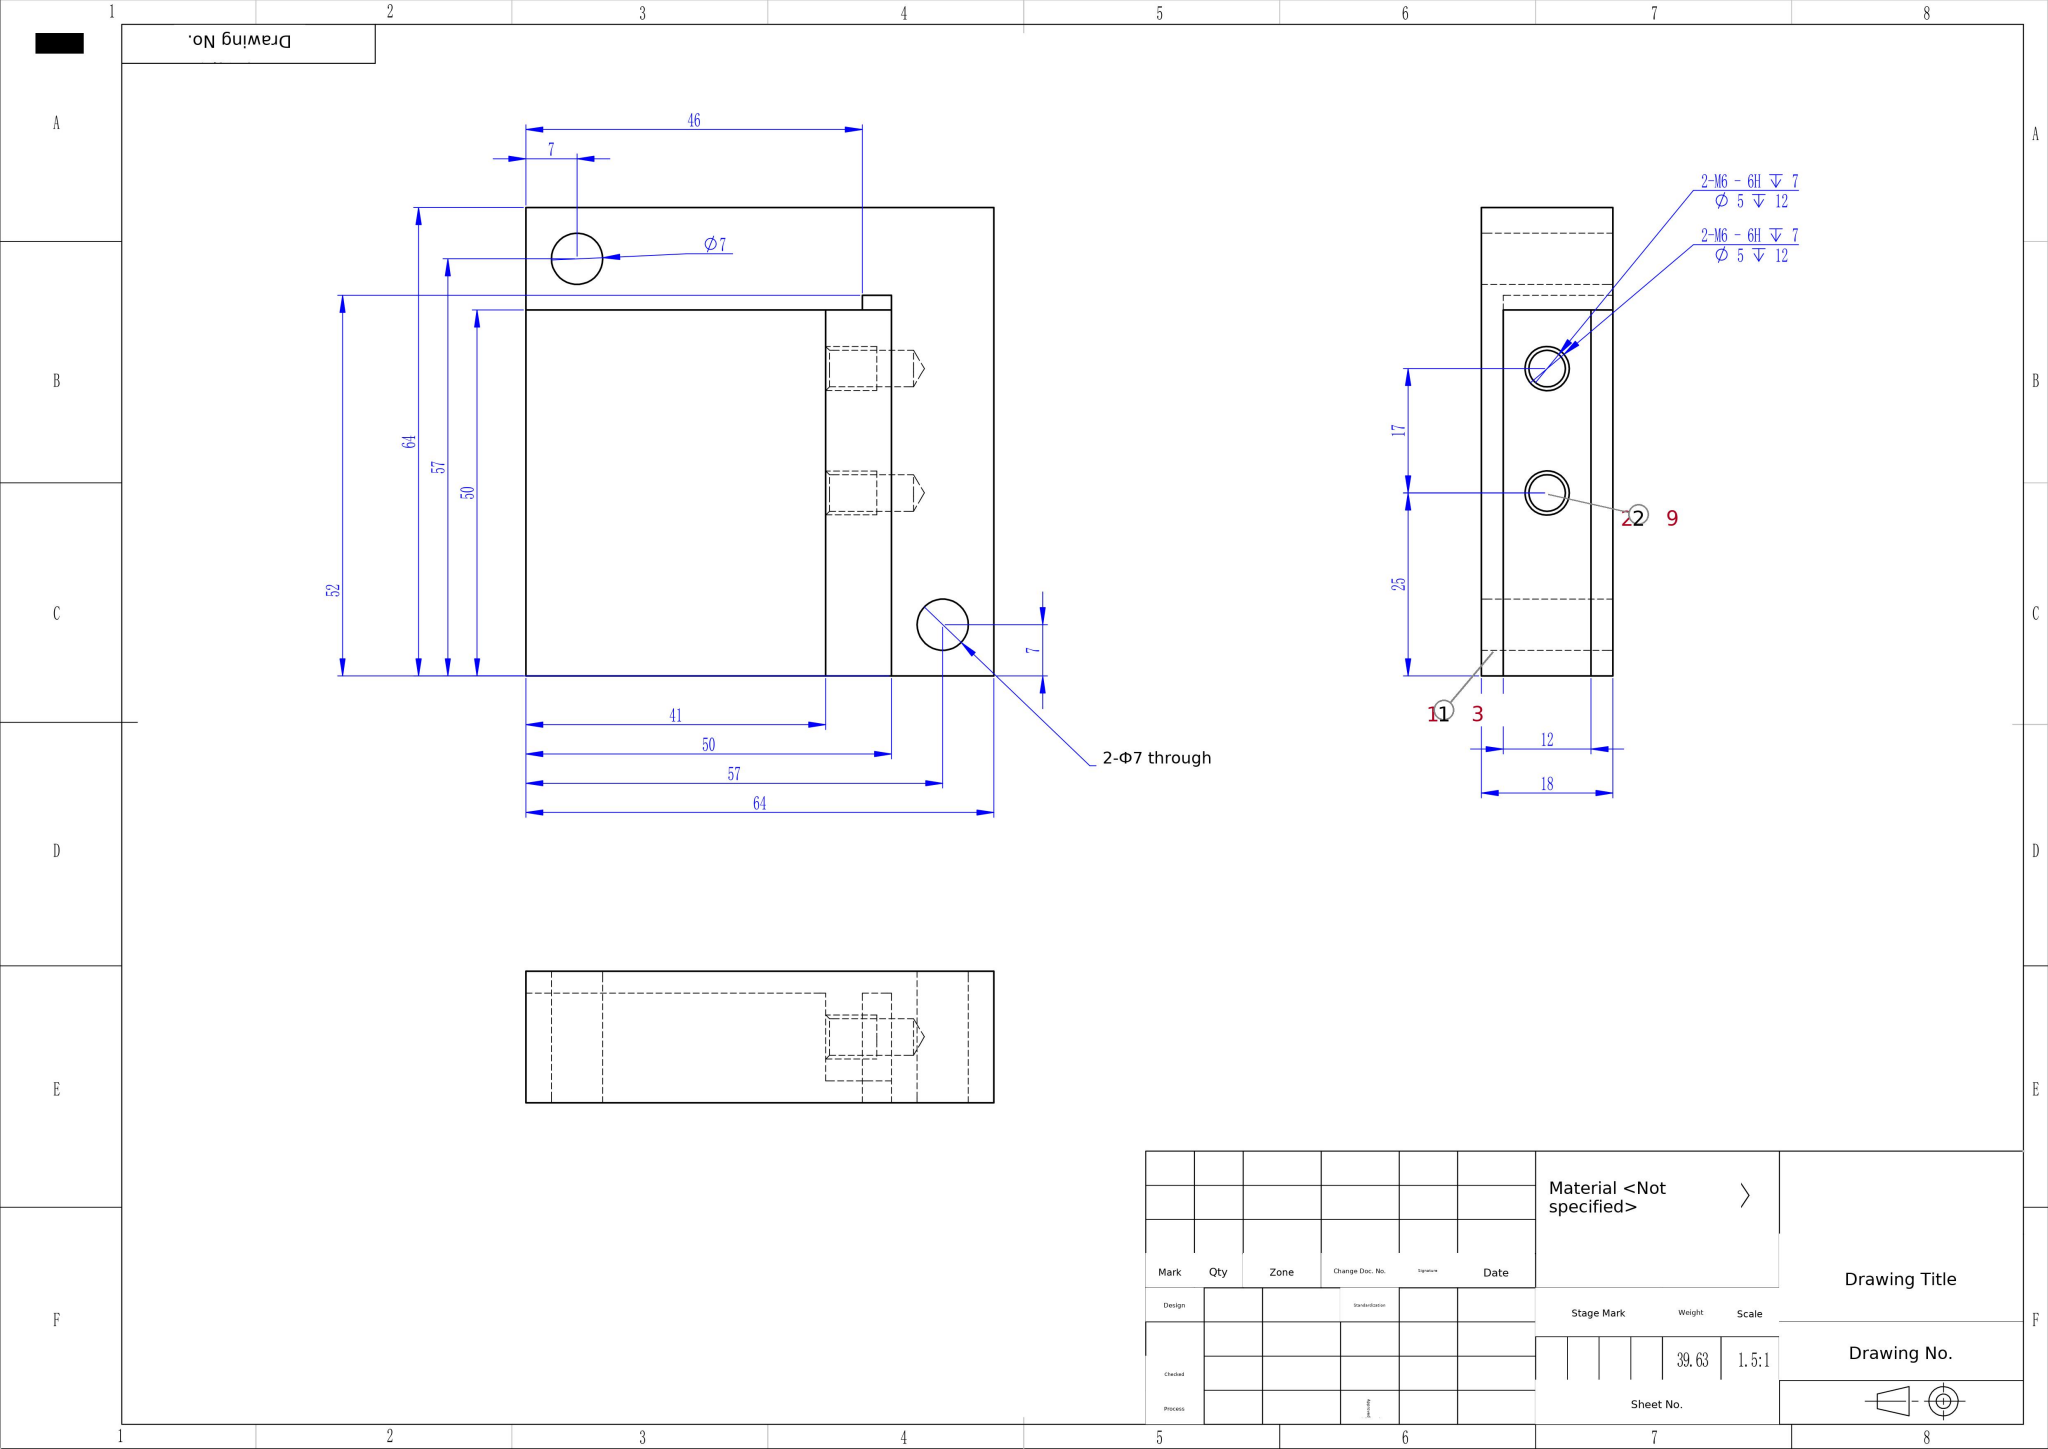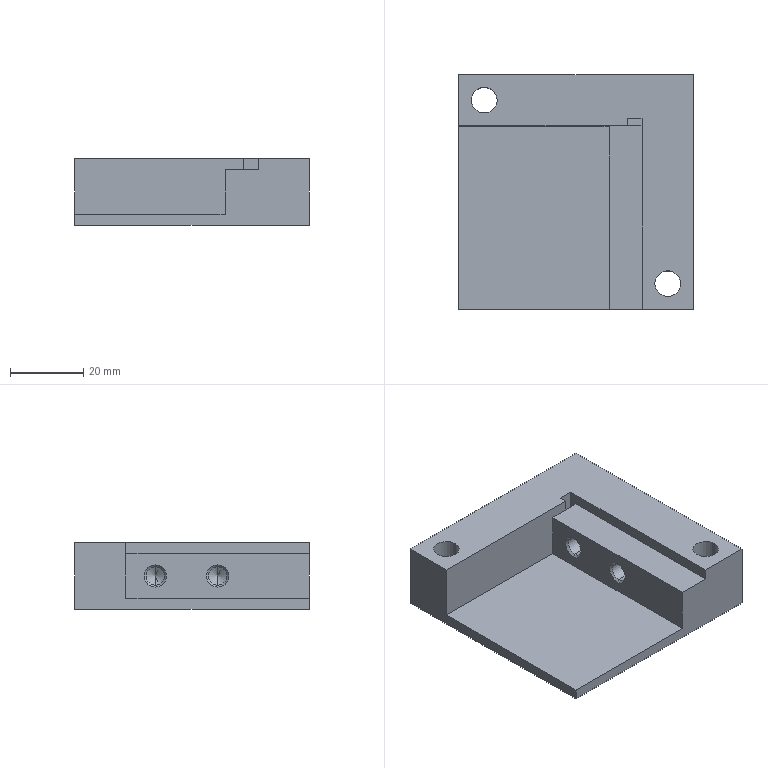Part | SolidWorks | mm | 1 solid | 31 faces | box 64 x 64 x 18 mm | volume 39627 mm3 | plane 15 | cone 8 | cylinder 8 | commonest cylinder face diameters 5 x4 7 x4
build123d program:
from build123d import *

# Parameters (mm, degrees)
SKETCH1_W                   = 64
SKETCH1_H                   = 64
BOSS_EXTRUDE1_DEPTH         = 3
BOSS_EXTRUDE2_DEPTH         = 15
CUT_EXTRUDE1_REACH          = 50.703
SKETCH4_R                   = 3.5
SKETCH6_W                   = 9
SKETCH6_H                   = 12
BOSS_EXTRUDE3_DEPTH         = 50
M6_TAPPED_HOLE1_D           = 5
M6_TAPPED_HOLE1_DEPTH       = 12
M6_TAPPED_HOLE1_CSINK_D     = 6.05
M6_TAPPED_HOLE1_CSINK_ANGLE = 90
M6_TAPPED_HOLE1_TIP         = 1.502


with BuildPart() as part:
    # Sketch1 → Boss-Extrude1 (new body)
    with BuildSketch(Plane.XY):
        Rectangle(SKETCH1_W, SKETCH1_H)
    extrude(amount=BOSS_EXTRUDE1_DEPTH)

    # Sketch3 → Boss-Extrude2 (add)
    with BuildSketch(Plane.XY.offset(3)):
        Polygon((-32, 32), (32, 32), (32, -32), (18, -32), (18, 20), (14, 20), (14, 18), (-32, 18), align=None)
    extrude(amount=BOSS_EXTRUDE2_DEPTH)

    # Sketch4 → Cut-Extrude1 (cut, up to next)
    with BuildSketch(Plane.XY.offset(18), mode=Mode.PRIVATE) as cut_extrude1_sk1:
        with Locations((-25, 25)):
            Circle(SKETCH4_R)
    cut_extrude1_tool1 = extrude(cut_extrude1_sk1.sketch, amount=-CUT_EXTRUDE1_REACH, mode=Mode.PRIVATE) & part.part
    # Sketch4 → Cut-Extrude1 (cut, up to next)
    with BuildSketch(Plane.XY.offset(18), mode=Mode.PRIVATE) as cut_extrude1_sk2:
        with Locations((25, -25)):
            Circle(SKETCH4_R)
    cut_extrude1_tool2 = extrude(cut_extrude1_sk2.sketch, amount=-CUT_EXTRUDE1_REACH, mode=Mode.PRIVATE) & part.part
    add(cut_extrude1_tool1.solids().sort_by_distance((-25, 25, 18))[0], mode=Mode.SUBTRACT)
    add(cut_extrude1_tool2.solids().sort_by_distance((25, -25, 18))[0], mode=Mode.SUBTRACT)

    # Sketch6 → Boss-Extrude3 (add)
    with BuildSketch(Plane.XZ.offset(32)):
        with Locations((13.5, 9)):
            Rectangle(SKETCH6_W, SKETCH6_H)
    extrude(amount=-BOSS_EXTRUDE3_DEPTH)

    # M6 Tapped Hole1
    with Locations(Plane.ZY.offset(-9)):
        with Locations((9, 10), (9, -7)):
            CounterSinkHole(M6_TAPPED_HOLE1_D / 2, M6_TAPPED_HOLE1_CSINK_D / 2, depth=M6_TAPPED_HOLE1_DEPTH, counter_sink_angle=M6_TAPPED_HOLE1_CSINK_ANGLE)
            with Locations((0, 0, -(M6_TAPPED_HOLE1_DEPTH + M6_TAPPED_HOLE1_TIP / 2))):  # 118° drill point
                Cone(0, M6_TAPPED_HOLE1_D / 2, M6_TAPPED_HOLE1_TIP, mode=Mode.SUBTRACT)


solid = part.part
STEP:
#1=CARTESIAN_POINT('',(9.525,10.,6.5));
#2=VERTEX_POINT('',#1);
#3=CARTESIAN_POINT('',(9.525,10.,11.5));
#4=VERTEX_POINT('',#3);
#5=CARTESIAN_POINT('',(9.525,10.,9.));
#6=DIRECTION('',(-1.,0.,-0.));
#7=DIRECTION('',(0.,0.,1.));
#8=AXIS2_PLACEMENT_3D('',#5,#6,#7);
#9=CIRCLE('',#8,2.5);
#10=EDGE_CURVE('',#2,#4,#9,.T.);
#11=ORIENTED_EDGE('',*,*,#10,.F.);
#12=CARTESIAN_POINT('',(9.,10.,5.975));
#13=VERTEX_POINT('',#12);
#14=CARTESIAN_POINT('',(9.,10.,5.975));
#15=DIRECTION('',(-0.7071,0.,-0.7071));
#16=VECTOR('',#15,1000.);
#17=LINE('',#14,#16);
#18=EDGE_CURVE('',#2,#13,#17,.T.);
#19=ORIENTED_EDGE('',*,*,#18,.T.);
#20=CARTESIAN_POINT('',(9.,10.,12.025));
#21=VERTEX_POINT('',#20);
#22=CARTESIAN_POINT('',(9.,10.,9.));
#23=DIRECTION('',(-1.,0.,-0.));
#24=DIRECTION('',(0.,0.,1.));
#25=AXIS2_PLACEMENT_3D('',#22,#23,#24);
#26=CIRCLE('',#25,3.025);
#27=EDGE_CURVE('',#13,#21,#26,.T.);
#28=ORIENTED_EDGE('',*,*,#27,.T.);
#29=CARTESIAN_POINT('',(9.,10.,12.025));
#30=DIRECTION('',(-0.7071,0.,0.7071));
#31=VECTOR('',#30,1000.);
#32=LINE('',#29,#31);
#33=EDGE_CURVE('',#4,#21,#32,.T.);
#34=ORIENTED_EDGE('',*,*,#33,.F.);
#35=EDGE_LOOP('',(#11,#19,#28,#34));
#36=FACE_OUTER_BOUND('',#35,.T.);
#37=CARTESIAN_POINT('',(9.,10.,9.));
#38=DIRECTION('',(-1.,0.,-0.));
#39=DIRECTION('',(0.,0.,1.));
#40=AXIS2_PLACEMENT_3D('',#37,#38,#39);
#41=CONICAL_SURFACE('',#40,3.025,0.7854);
#42=ADVANCED_FACE('',(#36),#41,.F.);
#43=CARTESIAN_POINT('',(21.,10.,6.5));
#44=VERTEX_POINT('',#43);
#45=CARTESIAN_POINT('',(21.,10.,11.5));
#46=VERTEX_POINT('',#45);
#47=CARTESIAN_POINT('',(21.,10.,9.));
#48=DIRECTION('',(-1.,0.,-0.));
#49=DIRECTION('',(0.,0.,1.));
#50=AXIS2_PLACEMENT_3D('',#47,#48,#49);
#51=CIRCLE('',#50,2.5);
#52=EDGE_CURVE('',#44,#46,#51,.T.);
#53=ORIENTED_EDGE('',*,*,#52,.F.);
#54=CARTESIAN_POINT('',(9.,10.,6.5));
#55=DIRECTION('',(-1.,0.,-0.));
#56=VECTOR('',#55,1000.);
#57=LINE('',#54,#56);
#58=EDGE_CURVE('',#44,#2,#57,.T.);
#59=ORIENTED_EDGE('',*,*,#58,.T.);
#60=ORIENTED_EDGE('',*,*,#10,.T.);
#61=CARTESIAN_POINT('',(9.,10.,11.5));
#62=DIRECTION('',(-1.,0.,-0.));
#63=VECTOR('',#62,1000.);
#64=LINE('',#61,#63);
#65=EDGE_CURVE('',#46,#4,#64,.T.);
#66=ORIENTED_EDGE('',*,*,#65,.F.);
#67=EDGE_LOOP('',(#53,#59,#60,#66));
#68=FACE_OUTER_BOUND('',#67,.T.);
#69=CARTESIAN_POINT('',(9.,10.,9.));
#70=DIRECTION('',(-1.,0.,-0.));
#71=DIRECTION('',(0.,0.,1.));
#72=AXIS2_PLACEMENT_3D('',#69,#70,#71);
#73=CYLINDRICAL_SURFACE('',#72,2.5);
#74=ADVANCED_FACE('',(#68),#73,.F.);
#75=CARTESIAN_POINT('',(22.502,10.,9.));
#76=VERTEX_POINT('',#75);
#77=CARTESIAN_POINT('',(21.,10.,11.5));
#78=DIRECTION('',(-0.515,0.,0.8572));
#79=VECTOR('',#78,1000.);
#80=LINE('',#77,#79);
#81=EDGE_CURVE('',#76,#46,#80,.T.);
#82=ORIENTED_EDGE('',*,*,#81,.F.);
#83=CARTESIAN_POINT('',(21.,10.,6.5));
#84=DIRECTION('',(-0.515,0.,-0.8572));
#85=VECTOR('',#84,1000.);
#86=LINE('',#83,#85);
#87=EDGE_CURVE('',#76,#44,#86,.T.);
#88=ORIENTED_EDGE('',*,*,#87,.T.);
#89=ORIENTED_EDGE('',*,*,#52,.T.);
#90=EDGE_LOOP('',(#82,#88,#89));
#91=FACE_OUTER_BOUND('',#90,.T.);
#92=CARTESIAN_POINT('',(21.,10.,9.));
#93=DIRECTION('',(-1.,0.,-0.));
#94=DIRECTION('',(0.,0.,1.));
#95=AXIS2_PLACEMENT_3D('',#92,#93,#94);
#96=CONICAL_SURFACE('',#95,2.5,1.03);
#97=ADVANCED_FACE('',(#91),#96,.F.);
#98=CARTESIAN_POINT('',(9.525,-7.,6.5));
#99=VERTEX_POINT('',#98);
#100=CARTESIAN_POINT('',(9.525,-7.,11.5));
#101=VERTEX_POINT('',#100);
#102=CARTESIAN_POINT('',(9.525,-7.,9.));
#103=DIRECTION('',(-1.,0.,-0.));
#104=DIRECTION('',(0.,0.,1.));
#105=AXIS2_PLACEMENT_3D('',#102,#103,#104);
#106=CIRCLE('',#105,2.5);
#107=EDGE_CURVE('',#99,#101,#106,.T.);
#108=ORIENTED_EDGE('',*,*,#107,.F.);
#109=CARTESIAN_POINT('',(9.,-7.,5.975));
#110=VERTEX_POINT('',#109);
#111=CARTESIAN_POINT('',(9.,-7.,5.975));
#112=DIRECTION('',(-0.7071,0.,-0.7071));
#113=VECTOR('',#112,1000.);
#114=LINE('',#111,#113);
#115=EDGE_CURVE('',#99,#110,#114,.T.);
#116=ORIENTED_EDGE('',*,*,#115,.T.);
#117=CARTESIAN_POINT('',(9.,-7.,12.025));
#118=VERTEX_POINT('',#117);
#119=CARTESIAN_POINT('',(9.,-7.,9.));
#120=DIRECTION('',(-1.,0.,-0.));
#121=DIRECTION('',(0.,0.,1.));
#122=AXIS2_PLACEMENT_3D('',#119,#120,#121);
#123=CIRCLE('',#122,3.025);
#124=EDGE_CURVE('',#110,#118,#123,.T.);
#125=ORIENTED_EDGE('',*,*,#124,.T.);
#126=CARTESIAN_POINT('',(9.,-7.,12.025));
#127=DIRECTION('',(-0.7071,0.,0.7071));
#128=VECTOR('',#127,1000.);
#129=LINE('',#126,#128);
#130=EDGE_CURVE('',#101,#118,#129,.T.);
#131=ORIENTED_EDGE('',*,*,#130,.F.);
#132=EDGE_LOOP('',(#108,#116,#125,#131));
#133=FACE_OUTER_BOUND('',#132,.T.);
#134=CARTESIAN_POINT('',(9.,-7.,9.));
#135=DIRECTION('',(-1.,0.,-0.));
#136=DIRECTION('',(0.,0.,1.));
#137=AXIS2_PLACEMENT_3D('',#134,#135,#136);
#138=CONICAL_SURFACE('',#137,3.025,0.7854);
#139=ADVANCED_FACE('',(#133),#138,.F.);
#140=CARTESIAN_POINT('',(21.,-7.,6.5));
#141=VERTEX_POINT('',#140);
#142=CARTESIAN_POINT('',(21.,-7.,11.5));
#143=VERTEX_POINT('',#142);
#144=CARTESIAN_POINT('',(21.,-7.,9.));
#145=DIRECTION('',(-1.,0.,-0.));
#146=DIRECTION('',(0.,0.,1.));
#147=AXIS2_PLACEMENT_3D('',#144,#145,#146);
#148=CIRCLE('',#147,2.5);
#149=EDGE_CURVE('',#141,#143,#148,.T.);
#150=ORIENTED_EDGE('',*,*,#149,.F.);
#151=CARTESIAN_POINT('',(9.,-7.,6.5));
#152=DIRECTION('',(-1.,0.,-0.));
#153=VECTOR('',#152,1000.);
#154=LINE('',#151,#153);
#155=EDGE_CURVE('',#141,#99,#154,.T.);
#156=ORIENTED_EDGE('',*,*,#155,.T.);
#157=ORIENTED_EDGE('',*,*,#107,.T.);
#158=CARTESIAN_POINT('',(9.,-7.,11.5));
#159=DIRECTION('',(-1.,0.,-0.));
#160=VECTOR('',#159,1000.);
#161=LINE('',#158,#160);
#162=EDGE_CURVE('',#143,#101,#161,.T.);
#163=ORIENTED_EDGE('',*,*,#162,.F.);
#164=EDGE_LOOP('',(#150,#156,#157,#163));
#165=FACE_OUTER_BOUND('',#164,.T.);
#166=CARTESIAN_POINT('',(9.,-7.,9.));
#167=DIRECTION('',(-1.,0.,-0.));
#168=DIRECTION('',(0.,0.,1.));
#169=AXIS2_PLACEMENT_3D('',#166,#167,#168);
#170=CYLINDRICAL_SURFACE('',#169,2.5);
#171=ADVANCED_FACE('',(#165),#170,.F.);
#172=CARTESIAN_POINT('',(22.502,-7.,9.));
#173=VERTEX_POINT('',#172);
#174=CARTESIAN_POINT('',(21.,-7.,11.5));
#175=DIRECTION('',(-0.515,0.,0.8572));
#176=VECTOR('',#175,1000.);
#177=LINE('',#174,#176);
#178=EDGE_CURVE('',#173,#143,#177,.T.);
#179=ORIENTED_EDGE('',*,*,#178,.F.);
#180=CARTESIAN_POINT('',(21.,-7.,6.5));
#181=DIRECTION('',(-0.515,0.,-0.8572));
#182=VECTOR('',#181,1000.);
#183=LINE('',#180,#182);
#184=EDGE_CURVE('',#173,#141,#183,.T.);
#185=ORIENTED_EDGE('',*,*,#184,.T.);
#186=ORIENTED_EDGE('',*,*,#149,.T.);
#187=EDGE_LOOP('',(#179,#185,#186));
#188=FACE_OUTER_BOUND('',#187,.T.);
#189=CARTESIAN_POINT('',(21.,-7.,9.));
#190=DIRECTION('',(-1.,0.,-0.));
#191=DIRECTION('',(0.,0.,1.));
#192=AXIS2_PLACEMENT_3D('',#189,#190,#191);
#193=CONICAL_SURFACE('',#192,2.5,1.03);
#194=ADVANCED_FACE('',(#188),#193,.F.);
#195=CARTESIAN_POINT('',(-28.5,25.,0.));
#196=VERTEX_POINT('',#195);
#197=CARTESIAN_POINT('',(-21.5,25.,0.));
#198=VERTEX_POINT('',#197);
#199=CARTESIAN_POINT('',(-25.,25.,0.));
#200=DIRECTION('',(0.,0.,1.));
#201=DIRECTION('',(-1.,0.,0.));
#202=AXIS2_PLACEMENT_3D('',#199,#200,#201);
#203=CIRCLE('',#202,3.5);
#204=EDGE_CURVE('',#196,#198,#203,.T.);
#205=ORIENTED_EDGE('',*,*,#204,.F.);
#206=CARTESIAN_POINT('',(-28.5,25.,18.));
#207=VERTEX_POINT('',#206);
#208=CARTESIAN_POINT('',(-28.5,25.,-0.001));
#209=DIRECTION('',(0.,0.,1.));
#210=VECTOR('',#209,1000.);
#211=LINE('',#208,#210);
#212=EDGE_CURVE('',#196,#207,#211,.T.);
#213=ORIENTED_EDGE('',*,*,#212,.T.);
#214=CARTESIAN_POINT('',(-21.5,25.,18.));
#215=VERTEX_POINT('',#214);
#216=CARTESIAN_POINT('',(-25.,25.,18.));
#217=DIRECTION('',(0.,0.,1.));
#218=DIRECTION('',(1.,0.,0.));
#219=AXIS2_PLACEMENT_3D('',#216,#217,#218);
#220=CIRCLE('',#219,3.5);
#221=EDGE_CURVE('',#207,#215,#220,.T.);
#222=ORIENTED_EDGE('',*,*,#221,.T.);
#223=CARTESIAN_POINT('',(-21.5,25.,-0.001));
#224=DIRECTION('',(0.,0.,1.));
#225=VECTOR('',#224,1000.);
#226=LINE('',#223,#225);
#227=EDGE_CURVE('',#198,#215,#226,.T.);
#228=ORIENTED_EDGE('',*,*,#227,.F.);
#229=EDGE_LOOP('',(#205,#213,#222,#228));
#230=FACE_OUTER_BOUND('',#229,.T.);
#231=CARTESIAN_POINT('',(-25.,25.,-0.001));
#232=DIRECTION('',(0.,0.,1.));
#233=DIRECTION('',(1.,0.,0.));
#234=AXIS2_PLACEMENT_3D('',#231,#232,#233);
#235=CYLINDRICAL_SURFACE('',#234,3.5);
#236=ADVANCED_FACE('',(#230),#235,.F.);
#237=CARTESIAN_POINT('',(21.5,-25.,0.));
#238=VERTEX_POINT('',#237);
#239=CARTESIAN_POINT('',(28.5,-25.,0.));
#240=VERTEX_POINT('',#239);
#241=CARTESIAN_POINT('',(25.,-25.,0.));
#242=DIRECTION('',(0.,0.,1.));
#243=DIRECTION('',(-1.,0.,0.));
#244=AXIS2_PLACEMENT_3D('',#241,#242,#243);
#245=CIRCLE('',#244,3.5);
#246=EDGE_CURVE('',#238,#240,#245,.T.);
#247=ORIENTED_EDGE('',*,*,#246,.F.);
#248=CARTESIAN_POINT('',(21.5,-25.,18.));
#249=VERTEX_POINT('',#248);
#250=CARTESIAN_POINT('',(21.5,-25.,-0.001));
#251=DIRECTION('',(0.,0.,1.));
#252=VECTOR('',#251,1000.);
#253=LINE('',#250,#252);
#254=EDGE_CURVE('',#238,#249,#253,.T.);
#255=ORIENTED_EDGE('',*,*,#254,.T.);
#256=CARTESIAN_POINT('',(28.5,-25.,18.));
#257=VERTEX_POINT('',#256);
#258=CARTESIAN_POINT('',(25.,-25.,18.));
#259=DIRECTION('',(0.,0.,1.));
#260=DIRECTION('',(1.,0.,0.));
#261=AXIS2_PLACEMENT_3D('',#258,#259,#260);
#262=CIRCLE('',#261,3.5);
#263=EDGE_CURVE('',#249,#257,#262,.T.);
#264=ORIENTED_EDGE('',*,*,#263,.T.);
#265=CARTESIAN_POINT('',(28.5,-25.,-0.001));
#266=DIRECTION('',(0.,0.,1.));
#267=VECTOR('',#266,1000.);
#268=LINE('',#265,#267);
#269=EDGE_CURVE('',#240,#257,#268,.T.);
#270=ORIENTED_EDGE('',*,*,#269,.F.);
#271=EDGE_LOOP('',(#247,#255,#264,#270));
#272=FACE_OUTER_BOUND('',#271,.T.);
#273=CARTESIAN_POINT('',(25.,-25.,-0.001));
#274=DIRECTION('',(0.,0.,1.));
#275=DIRECTION('',(1.,0.,0.));
#276=AXIS2_PLACEMENT_3D('',#273,#274,#275);
#277=CYLINDRICAL_SURFACE('',#276,3.5);
#278=ADVANCED_FACE('',(#272),#277,.F.);
#279=CARTESIAN_POINT('',(14.,18.,3.));
#280=VERTEX_POINT('',#279);
#281=CARTESIAN_POINT('',(14.,20.,3.));
#282=VERTEX_POINT('',#281);
#283=CARTESIAN_POINT('',(14.,20.,3.));
#284=DIRECTION('',(0.,1.,0.));
#285=VECTOR('',#284,1000.);
#286=LINE('',#283,#285);
#287=EDGE_CURVE('',#280,#282,#286,.T.);
#288=ORIENTED_EDGE('',*,*,#287,.F.);
#289=CARTESIAN_POINT('',(18.,18.,3.));
#290=VERTEX_POINT('',#289);
#291=CARTESIAN_POINT('',(9.,18.,3.));
#292=DIRECTION('',(1.,0.,0.));
#293=VECTOR('',#292,1000.);
#294=LINE('',#291,#293);
#295=EDGE_CURVE('',#280,#290,#294,.T.);
#296=ORIENTED_EDGE('',*,*,#295,.T.);
#297=CARTESIAN_POINT('',(18.,20.,3.));
#298=VERTEX_POINT('',#297);
#299=CARTESIAN_POINT('',(18.,-32.,3.));
#300=DIRECTION('',(0.,-1.,0.));
#301=VECTOR('',#300,1000.);
#302=LINE('',#299,#301);
#303=EDGE_CURVE('',#298,#290,#302,.T.);
#304=ORIENTED_EDGE('',*,*,#303,.F.);
#305=CARTESIAN_POINT('',(18.,20.,3.));
#306=DIRECTION('',(1.,-0.,0.));
#307=VECTOR('',#306,1000.);
#308=LINE('',#305,#307);
#309=EDGE_CURVE('',#282,#298,#308,.T.);
#310=ORIENTED_EDGE('',*,*,#309,.F.);
#311=EDGE_LOOP('',(#288,#296,#304,#310));
#312=FACE_OUTER_BOUND('',#311,.T.);
#313=CARTESIAN_POINT('',(0.,0.,3.));
#314=DIRECTION('',(0.,0.,-1.));
#315=DIRECTION('',(-1.,0.,0.));
#316=AXIS2_PLACEMENT_3D('',#313,#314,#315);
#317=PLANE('',#316);
#318=ADVANCED_FACE('',(#312),#317,.F.);
#319=CARTESIAN_POINT('',(-32.,-32.,3.));
#320=VERTEX_POINT('',#319);
#321=CARTESIAN_POINT('',(9.,-32.,3.));
#322=VERTEX_POINT('',#321);
#323=CARTESIAN_POINT('',(-32.,-32.,3.));
#324=DIRECTION('',(1.,0.,0.));
#325=VECTOR('',#324,1000.);
#326=LINE('',#323,#325);
#327=EDGE_CURVE('',#320,#322,#326,.T.);
#328=ORIENTED_EDGE('',*,*,#327,.T.);
#329=CARTESIAN_POINT('',(9.,18.,3.));
#330=VERTEX_POINT('',#329);
#331=CARTESIAN_POINT('',(9.,33.,3.));
#332=DIRECTION('',(0.,-1.,0.));
#333=VECTOR('',#332,1000.);
#334=LINE('',#331,#333);
#335=EDGE_CURVE('',#330,#322,#334,.T.);
#336=ORIENTED_EDGE('',*,*,#335,.F.);
#337=CARTESIAN_POINT('',(-32.,18.,3.));
#338=VERTEX_POINT('',#337);
#339=CARTESIAN_POINT('',(14.,18.,3.));
#340=DIRECTION('',(1.,0.,0.));
#341=VECTOR('',#340,1000.);
#342=LINE('',#339,#341);
#343=EDGE_CURVE('',#338,#330,#342,.T.);
#344=ORIENTED_EDGE('',*,*,#343,.F.);
#345=CARTESIAN_POINT('',(-32.,-32.,3.));
#346=DIRECTION('',(0.,-1.,0.));
#347=VECTOR('',#346,1000.);
#348=LINE('',#345,#347);
#349=EDGE_CURVE('',#338,#320,#348,.T.);
#350=ORIENTED_EDGE('',*,*,#349,.T.);
#351=EDGE_LOOP('',(#328,#336,#344,#350));
#352=FACE_OUTER_BOUND('',#351,.T.);
#353=CARTESIAN_POINT('',(0.,0.,3.));
#354=DIRECTION('',(0.,0.,-1.));
#355=DIRECTION('',(-1.,0.,0.));
#356=AXIS2_PLACEMENT_3D('',#353,#354,#355);
#357=PLANE('',#356);
#358=ADVANCED_FACE('',(#352),#357,.F.);
#359=CARTESIAN_POINT('',(32.,-32.,0.));
#360=VERTEX_POINT('',#359);
#361=CARTESIAN_POINT('',(32.,32.,0.));
#362=VERTEX_POINT('',#361);
#363=CARTESIAN_POINT('',(32.,-32.,0.));
#364=DIRECTION('',(0.,1.,0.));
#365=VECTOR('',#364,1000.);
#366=LINE('',#363,#365);
#367=EDGE_CURVE('',#360,#362,#366,.T.);
#368=ORIENTED_EDGE('',*,*,#367,.T.);
#369=CARTESIAN_POINT('',(32.,32.,18.));
#370=VERTEX_POINT('',#369);
#371=CARTESIAN_POINT('',(32.,32.,3.));
#372=DIRECTION('',(0.,0.,-1.));
#373=VECTOR('',#372,1000.);
#374=LINE('',#371,#373);
#375=EDGE_CURVE('',#370,#362,#374,.T.);
#376=ORIENTED_EDGE('',*,*,#375,.F.);
#377=CARTESIAN_POINT('',(32.,-32.,18.));
#378=VERTEX_POINT('',#377);
#379=CARTESIAN_POINT('',(32.,32.,18.));
#380=DIRECTION('',(0.,1.,0.));
#381=VECTOR('',#380,1000.);
#382=LINE('',#379,#381);
#383=EDGE_CURVE('',#378,#370,#382,.T.);
#384=ORIENTED_EDGE('',*,*,#383,.F.);
#385=CARTESIAN_POINT('',(32.,-32.,3.));
#386=DIRECTION('',(0.,0.,-1.));
#387=VECTOR('',#386,1000.);
#388=LINE('',#385,#387);
#389=EDGE_CURVE('',#378,#360,#388,.T.);
#390=ORIENTED_EDGE('',*,*,#389,.T.);
#391=EDGE_LOOP('',(#368,#376,#384,#390));
#392=FACE_OUTER_BOUND('',#391,.T.);
#393=CARTESIAN_POINT('',(32.,-32.,3.));
#394=DIRECTION('',(-1.,0.,0.));
#395=DIRECTION('',(0.,0.,1.));
#396=AXIS2_PLACEMENT_3D('',#393,#394,#395);
#397=PLANE('',#396);
#398=ADVANCED_FACE('',(#392),#397,.F.);
#399=CARTESIAN_POINT('',(-32.,32.,0.));
#400=VERTEX_POINT('',#399);
#401=CARTESIAN_POINT('',(-32.,32.,0.));
#402=DIRECTION('',(-1.,0.,0.));
#403=VECTOR('',#402,1000.);
#404=LINE('',#401,#403);
#405=EDGE_CURVE('',#362,#400,#404,.T.);
#406=ORIENTED_EDGE('',*,*,#405,.T.);
#407=CARTESIAN_POINT('',(-32.,32.,18.));
#408=VERTEX_POINT('',#407);
#409=CARTESIAN_POINT('',(-32.,32.,3.));
#410=DIRECTION('',(0.,0.,-1.));
#411=VECTOR('',#410,1000.);
#412=LINE('',#409,#411);
#413=EDGE_CURVE('',#408,#400,#412,.T.);
#414=ORIENTED_EDGE('',*,*,#413,.F.);
#415=CARTESIAN_POINT('',(-32.,32.,18.));
#416=DIRECTION('',(-1.,0.,0.));
#417=VECTOR('',#416,1000.);
#418=LINE('',#415,#417);
#419=EDGE_CURVE('',#370,#408,#418,.T.);
#420=ORIENTED_EDGE('',*,*,#419,.F.);
#421=ORIENTED_EDGE('',*,*,#375,.T.);
#422=EDGE_LOOP('',(#406,#414,#420,#421));
#423=FACE_OUTER_BOUND('',#422,.T.);
#424=CARTESIAN_POINT('',(-32.,32.,3.));
#425=DIRECTION('',(0.,-1.,0.));
#426=DIRECTION('',(0.,0.,-1.));
#427=AXIS2_PLACEMENT_3D('',#424,#425,#426);
#428=PLANE('',#427);
#429=ADVANCED_FACE('',(#423),#428,.F.);
#430=CARTESIAN_POINT('',(-32.,-32.,0.));
#431=VERTEX_POINT('',#430);
#432=CARTESIAN_POINT('',(-32.,-32.,0.));
#433=DIRECTION('',(0.,-1.,0.));
#434=VECTOR('',#433,1000.);
#435=LINE('',#432,#434);
#436=EDGE_CURVE('',#400,#431,#435,.T.);
#437=ORIENTED_EDGE('',*,*,#436,.T.);
#438=CARTESIAN_POINT('',(-32.,-32.,3.));
#439=DIRECTION('',(0.,0.,-1.));
#440=VECTOR('',#439,1000.);
#441=LINE('',#438,#440);
#442=EDGE_CURVE('',#320,#431,#441,.T.);
#443=ORIENTED_EDGE('',*,*,#442,.F.);
#444=ORIENTED_EDGE('',*,*,#349,.F.);
#445=CARTESIAN_POINT('',(-32.,18.,18.));
#446=VERTEX_POINT('',#445);
#447=CARTESIAN_POINT('',(-32.,18.,18.));
#448=DIRECTION('',(0.,0.,-1.));
#449=VECTOR('',#448,1000.);
#450=LINE('',#447,#449);
#451=EDGE_CURVE('',#446,#338,#450,.T.);
#452=ORIENTED_EDGE('',*,*,#451,.F.);
#453=CARTESIAN_POINT('',(-32.,18.,18.));
#454=DIRECTION('',(0.,-1.,0.));
#455=VECTOR('',#454,1000.);
#456=LINE('',#453,#455);
#457=EDGE_CURVE('',#408,#446,#456,.T.);
#458=ORIENTED_EDGE('',*,*,#457,.F.);
#459=ORIENTED_EDGE('',*,*,#413,.T.);
#460=EDGE_LOOP('',(#437,#443,#444,#452,#458,#459));
#461=FACE_OUTER_BOUND('',#460,.T.);
#462=CARTESIAN_POINT('',(-32.,-32.,3.));
#463=DIRECTION('',(1.,0.,0.));
#464=DIRECTION('',(0.,0.,-1.));
#465=AXIS2_PLACEMENT_3D('',#462,#463,#464);
#466=PLANE('',#465);
#467=ADVANCED_FACE('',(#461),#466,.F.);
#468=CARTESIAN_POINT('',(-32.,-32.,0.));
#469=DIRECTION('',(1.,0.,0.));
#470=VECTOR('',#469,1000.);
#471=LINE('',#468,#470);
#472=EDGE_CURVE('',#431,#360,#471,.T.);
#473=ORIENTED_EDGE('',*,*,#472,.T.);
#474=ORIENTED_EDGE('',*,*,#389,.F.);
#475=CARTESIAN_POINT('',(18.,-32.,18.));
#476=VERTEX_POINT('',#475);
#477=CARTESIAN_POINT('',(32.,-32.,18.));
#478=DIRECTION('',(1.,0.,0.));
#479=VECTOR('',#478,1000.);
#480=LINE('',#477,#479);
#481=EDGE_CURVE('',#476,#378,#480,.T.);
#482=ORIENTED_EDGE('',*,*,#481,.F.);
#483=CARTESIAN_POINT('',(18.,-32.,15.));
#484=VERTEX_POINT('',#483);
#485=CARTESIAN_POINT('',(18.,-32.,18.));
#486=DIRECTION('',(0.,0.,-1.));
#487=VECTOR('',#486,1000.);
#488=LINE('',#485,#487);
#489=EDGE_CURVE('',#476,#484,#488,.T.);
#490=ORIENTED_EDGE('',*,*,#489,.T.);
#491=CARTESIAN_POINT('',(9.,-32.,15.));
#492=VERTEX_POINT('',#491);
#493=CARTESIAN_POINT('',(18.,-32.,15.));
#494=DIRECTION('',(-1.,0.,-0.));
#495=VECTOR('',#494,1000.);
#496=LINE('',#493,#495);
#497=EDGE_CURVE('',#484,#492,#496,.T.);
#498=ORIENTED_EDGE('',*,*,#497,.T.);
#499=CARTESIAN_POINT('',(9.,-32.,15.));
#500=DIRECTION('',(0.,0.,-1.));
#501=VECTOR('',#500,1000.);
#502=LINE('',#499,#501);
#503=EDGE_CURVE('',#492,#322,#502,.T.);
#504=ORIENTED_EDGE('',*,*,#503,.T.);
#505=ORIENTED_EDGE('',*,*,#327,.F.);
#506=ORIENTED_EDGE('',*,*,#442,.T.);
#507=EDGE_LOOP('',(#473,#474,#482,#490,#498,#504,#505,#506));
#508=FACE_OUTER_BOUND('',#507,.T.);
#509=CARTESIAN_POINT('',(-32.,-32.,3.));
#510=DIRECTION('',(0.,1.,0.));
#511=DIRECTION('',(0.,0.,1.));
#512=AXIS2_PLACEMENT_3D('',#509,#510,#511);
#513=PLANE('',#512);
#514=ADVANCED_FACE('',(#508),#513,.F.);
#515=CARTESIAN_POINT('',(-25.,25.,0.));
#516=DIRECTION('',(0.,0.,1.));
#517=DIRECTION('',(-1.,0.,0.));
#518=AXIS2_PLACEMENT_3D('',#515,#516,#517);
#519=CIRCLE('',#518,3.5);
#520=EDGE_CURVE('',#198,#196,#519,.T.);
#521=ORIENTED_EDGE('',*,*,#520,.T.);
#522=ORIENTED_EDGE('',*,*,#204,.T.);
#523=EDGE_LOOP('',(#521,#522));
#524=FACE_BOUND('',#523,.T.);
#525=CARTESIAN_POINT('',(25.,-25.,0.));
#526=DIRECTION('',(0.,0.,1.));
#527=DIRECTION('',(-1.,0.,0.));
#528=AXIS2_PLACEMENT_3D('',#525,#526,#527);
#529=CIRCLE('',#528,3.5);
#530=EDGE_CURVE('',#240,#238,#529,.T.);
#531=ORIENTED_EDGE('',*,*,#530,.T.);
#532=ORIENTED_EDGE('',*,*,#246,.T.);
#533=EDGE_LOOP('',(#531,#532));
#534=FACE_BOUND('',#533,.T.);
#535=ORIENTED_EDGE('',*,*,#367,.F.);
#536=ORIENTED_EDGE('',*,*,#472,.F.);
#537=ORIENTED_EDGE('',*,*,#436,.F.);
#538=ORIENTED_EDGE('',*,*,#405,.F.);
#539=EDGE_LOOP('',(#535,#536,#537,#538));
#540=FACE_OUTER_BOUND('',#539,.T.);
#541=CARTESIAN_POINT('',(0.,0.,0.));
#542=DIRECTION('',(0.,0.,-1.));
#543=DIRECTION('',(-1.,0.,0.));
#544=AXIS2_PLACEMENT_3D('',#541,#542,#543);
#545=PLANE('',#544);
#546=ADVANCED_FACE('',(#524,#534,#540),#545,.T.);
#547=CARTESIAN_POINT('',(9.,18.,15.));
#548=VERTEX_POINT('',#547);
#549=CARTESIAN_POINT('',(9.,18.,15.));
#550=DIRECTION('',(0.,0.,-1.));
#551=VECTOR('',#550,1000.);
#552=LINE('',#549,#551);
#553=EDGE_CURVE('',#548,#330,#552,.T.);
#554=ORIENTED_EDGE('',*,*,#553,.F.);
#555=CARTESIAN_POINT('',(14.,18.,15.));
#556=VERTEX_POINT('',#555);
#557=CARTESIAN_POINT('',(18.,18.,15.));
#558=DIRECTION('',(-1.,0.,-0.));
#559=VECTOR('',#558,1000.);
#560=LINE('',#557,#559);
#561=EDGE_CURVE('',#556,#548,#560,.T.);
#562=ORIENTED_EDGE('',*,*,#561,.F.);
#563=CARTESIAN_POINT('',(14.,18.,18.));
#564=VERTEX_POINT('',#563);
#565=CARTESIAN_POINT('',(14.,18.,18.));
#566=DIRECTION('',(0.,0.,-1.));
#567=VECTOR('',#566,1000.);
#568=LINE('',#565,#567);
#569=EDGE_CURVE('',#564,#556,#568,.T.);
#570=ORIENTED_EDGE('',*,*,#569,.F.);
#571=CARTESIAN_POINT('',(14.,18.,18.));
#572=DIRECTION('',(1.,0.,0.));
#573=VECTOR('',#572,1000.);
#574=LINE('',#571,#573);
#575=EDGE_CURVE('',#446,#564,#574,.T.);
#576=ORIENTED_EDGE('',*,*,#575,.F.);
#577=ORIENTED_EDGE('',*,*,#451,.T.);
#578=ORIENTED_EDGE('',*,*,#343,.T.);
#579=EDGE_LOOP('',(#554,#562,#570,#576,#577,#578));
#580=FACE_OUTER_BOUND('',#579,.T.);
#581=CARTESIAN_POINT('',(14.,18.,18.));
#582=DIRECTION('',(0.,1.,0.));
#583=DIRECTION('',(0.,0.,1.));
#584=AXIS2_PLACEMENT_3D('',#581,#582,#583);
#585=PLANE('',#584);
#586=ADVANCED_FACE('',(#580),#585,.F.);
#587=ORIENTED_EDGE('',*,*,#287,.T.);
#588=CARTESIAN_POINT('',(14.,20.,18.));
#589=VERTEX_POINT('',#588);
#590=CARTESIAN_POINT('',(14.,20.,18.));
#591=DIRECTION('',(0.,0.,-1.));
#592=VECTOR('',#591,1000.);
#593=LINE('',#590,#592);
#594=EDGE_CURVE('',#589,#282,#593,.T.);
#595=ORIENTED_EDGE('',*,*,#594,.F.);
#596=CARTESIAN_POINT('',(14.,20.,18.));
#597=DIRECTION('',(0.,1.,0.));
#598=VECTOR('',#597,1000.);
#599=LINE('',#596,#598);
#600=EDGE_CURVE('',#564,#589,#599,.T.);
#601=ORIENTED_EDGE('',*,*,#600,.F.);
#602=ORIENTED_EDGE('',*,*,#569,.T.);
#603=CARTESIAN_POINT('',(14.,18.,18.));
#604=DIRECTION('',(0.,0.,-1.));
#605=VECTOR('',#604,1000.);
#606=LINE('',#603,#605);
#607=EDGE_CURVE('',#556,#280,#606,.T.);
#608=ORIENTED_EDGE('',*,*,#607,.T.);
#609=EDGE_LOOP('',(#587,#595,#601,#602,#608));
#610=FACE_OUTER_BOUND('',#609,.T.);
#611=CARTESIAN_POINT('',(14.,20.,18.));
#612=DIRECTION('',(-1.,0.,0.));
#613=DIRECTION('',(0.,0.,1.));
#614=AXIS2_PLACEMENT_3D('',#611,#612,#613);
#615=PLANE('',#614);
#616=ADVANCED_FACE('',(#610),#615,.F.);
#617=ORIENTED_EDGE('',*,*,#309,.T.);
#618=CARTESIAN_POINT('',(18.,20.,18.));
#619=VERTEX_POINT('',#618);
#620=CARTESIAN_POINT('',(18.,20.,18.));
#621=DIRECTION('',(0.,0.,-1.));
#622=VECTOR('',#621,1000.);
#623=LINE('',#620,#622);
#624=EDGE_CURVE('',#619,#298,#623,.T.);
#625=ORIENTED_EDGE('',*,*,#624,.F.);
#626=CARTESIAN_POINT('',(18.,20.,18.));
#627=DIRECTION('',(1.,-0.,0.));
#628=VECTOR('',#627,1000.);
#629=LINE('',#626,#628);
#630=EDGE_CURVE('',#589,#619,#629,.T.);
#631=ORIENTED_EDGE('',*,*,#630,.F.);
#632=ORIENTED_EDGE('',*,*,#594,.T.);
#633=EDGE_LOOP('',(#617,#625,#631,#632));
#634=FACE_OUTER_BOUND('',#633,.T.);
#635=CARTESIAN_POINT('',(18.,20.,18.));
#636=DIRECTION('',(0.,1.,0.));
#637=DIRECTION('',(-1.,0.,0.));
#638=AXIS2_PLACEMENT_3D('',#635,#636,#637);
#639=PLANE('',#638);
#640=ADVANCED_FACE('',(#634),#639,.F.);
#641=ORIENTED_EDGE('',*,*,#303,.T.);
#642=CARTESIAN_POINT('',(18.,18.,15.));
#643=VERTEX_POINT('',#642);
#644=CARTESIAN_POINT('',(18.,18.,3.));
#645=DIRECTION('',(0.,0.,1.));
#646=VECTOR('',#645,1000.);
#647=LINE('',#644,#646);
#648=EDGE_CURVE('',#290,#643,#647,.T.);
#649=ORIENTED_EDGE('',*,*,#648,.T.);
#650=CARTESIAN_POINT('',(18.,33.,15.));
#651=DIRECTION('',(0.,-1.,0.));
#652=VECTOR('',#651,1000.);
#653=LINE('',#650,#652);
#654=EDGE_CURVE('',#643,#484,#653,.T.);
#655=ORIENTED_EDGE('',*,*,#654,.T.);
#656=ORIENTED_EDGE('',*,*,#489,.F.);
#657=CARTESIAN_POINT('',(18.,-32.,18.));
#658=DIRECTION('',(0.,-1.,0.));
#659=VECTOR('',#658,1000.);
#660=LINE('',#657,#659);
#661=EDGE_CURVE('',#619,#476,#660,.T.);
#662=ORIENTED_EDGE('',*,*,#661,.F.);
#663=ORIENTED_EDGE('',*,*,#624,.T.);
#664=EDGE_LOOP('',(#641,#649,#655,#656,#662,#663));
#665=FACE_OUTER_BOUND('',#664,.T.);
#666=CARTESIAN_POINT('',(18.,-32.,18.));
#667=DIRECTION('',(1.,0.,0.));
#668=DIRECTION('',(0.,0.,-1.));
#669=AXIS2_PLACEMENT_3D('',#666,#667,#668);
#670=PLANE('',#669);
#671=ADVANCED_FACE('',(#665),#670,.F.);
#672=CARTESIAN_POINT('',(-25.,25.,18.));
#673=DIRECTION('',(0.,0.,1.));
#674=DIRECTION('',(1.,0.,0.));
#675=AXIS2_PLACEMENT_3D('',#672,#673,#674);
#676=CIRCLE('',#675,3.5);
#677=EDGE_CURVE('',#215,#207,#676,.T.);
#678=ORIENTED_EDGE('',*,*,#677,.F.);
#679=ORIENTED_EDGE('',*,*,#221,.F.);
#680=EDGE_LOOP('',(#678,#679));
#681=FACE_BOUND('',#680,.T.);
#682=CARTESIAN_POINT('',(25.,-25.,18.));
#683=DIRECTION('',(0.,0.,1.));
#684=DIRECTION('',(1.,0.,0.));
#685=AXIS2_PLACEMENT_3D('',#682,#683,#684);
#686=CIRCLE('',#685,3.5);
#687=EDGE_CURVE('',#257,#249,#686,.T.);
#688=ORIENTED_EDGE('',*,*,#687,.F.);
#689=ORIENTED_EDGE('',*,*,#263,.F.);
#690=EDGE_LOOP('',(#688,#689));
#691=FACE_BOUND('',#690,.T.);
#692=ORIENTED_EDGE('',*,*,#457,.T.);
#693=ORIENTED_EDGE('',*,*,#575,.T.);
#694=ORIENTED_EDGE('',*,*,#600,.T.);
#695=ORIENTED_EDGE('',*,*,#630,.T.);
#696=ORIENTED_EDGE('',*,*,#661,.T.);
#697=ORIENTED_EDGE('',*,*,#481,.T.);
#698=ORIENTED_EDGE('',*,*,#383,.T.);
#699=ORIENTED_EDGE('',*,*,#419,.T.);
#700=EDGE_LOOP('',(#692,#693,#694,#695,#696,#697,#698,#699));
#701=FACE_OUTER_BOUND('',#700,.T.);
#702=CARTESIAN_POINT('',(0.,0.,18.));
#703=DIRECTION('',(0.,0.,-1.));
#704=DIRECTION('',(-1.,0.,0.));
#705=AXIS2_PLACEMENT_3D('',#702,#703,#704);
#706=PLANE('',#705);
#707=ADVANCED_FACE('',(#681,#691,#701),#706,.F.);
#708=ORIENTED_EDGE('',*,*,#254,.F.);
#709=ORIENTED_EDGE('',*,*,#530,.F.);
#710=ORIENTED_EDGE('',*,*,#269,.T.);
#711=ORIENTED_EDGE('',*,*,#687,.T.);
#712=EDGE_LOOP('',(#708,#709,#710,#711));
#713=FACE_OUTER_BOUND('',#712,.T.);
#714=CARTESIAN_POINT('',(25.,-25.,-0.001));
#715=DIRECTION('',(0.,0.,1.));
#716=DIRECTION('',(1.,0.,0.));
#717=AXIS2_PLACEMENT_3D('',#714,#715,#716);
#718=CYLINDRICAL_SURFACE('',#717,3.5);
#719=ADVANCED_FACE('',(#713),#718,.F.);
#720=ORIENTED_EDGE('',*,*,#212,.F.);
#721=ORIENTED_EDGE('',*,*,#520,.F.);
#722=ORIENTED_EDGE('',*,*,#227,.T.);
#723=ORIENTED_EDGE('',*,*,#677,.T.);
#724=EDGE_LOOP('',(#720,#721,#722,#723));
#725=FACE_OUTER_BOUND('',#724,.T.);
#726=CARTESIAN_POINT('',(-25.,25.,-0.001));
#727=DIRECTION('',(0.,0.,1.));
#728=DIRECTION('',(1.,0.,0.));
#729=AXIS2_PLACEMENT_3D('',#726,#727,#728);
#730=CYLINDRICAL_SURFACE('',#729,3.5);
#731=ADVANCED_FACE('',(#725),#730,.F.);
#732=ORIENTED_EDGE('',*,*,#607,.F.);
#733=CARTESIAN_POINT('',(18.,18.,15.));
#734=DIRECTION('',(-1.,0.,-0.));
#735=VECTOR('',#734,1000.);
#736=LINE('',#733,#735);
#737=EDGE_CURVE('',#643,#556,#736,.T.);
#738=ORIENTED_EDGE('',*,*,#737,.F.);
#739=ORIENTED_EDGE('',*,*,#648,.F.);
#740=ORIENTED_EDGE('',*,*,#295,.F.);
#741=EDGE_LOOP('',(#732,#738,#739,#740));
#742=FACE_OUTER_BOUND('',#741,.T.);
#743=CARTESIAN_POINT('',(14.,18.,18.));
#744=DIRECTION('',(0.,1.,0.));
#745=DIRECTION('',(0.,0.,1.));
#746=AXIS2_PLACEMENT_3D('',#743,#744,#745);
#747=PLANE('',#746);
#748=ADVANCED_FACE('',(#742),#747,.T.);
#749=ORIENTED_EDGE('',*,*,#654,.F.);
#750=ORIENTED_EDGE('',*,*,#737,.T.);
#751=ORIENTED_EDGE('',*,*,#561,.T.);
#752=CARTESIAN_POINT('',(9.,33.,15.));
#753=DIRECTION('',(0.,-1.,0.));
#754=VECTOR('',#753,1000.);
#755=LINE('',#752,#754);
#756=EDGE_CURVE('',#548,#492,#755,.T.);
#757=ORIENTED_EDGE('',*,*,#756,.T.);
#758=ORIENTED_EDGE('',*,*,#497,.F.);
#759=EDGE_LOOP('',(#749,#750,#751,#757,#758));
#760=FACE_OUTER_BOUND('',#759,.T.);
#761=CARTESIAN_POINT('',(18.,33.,15.));
#762=DIRECTION('',(-0.,0.,1.));
#763=DIRECTION('',(1.,0.,0.));
#764=AXIS2_PLACEMENT_3D('',#761,#762,#763);
#765=PLANE('',#764);
#766=ADVANCED_FACE('',(#760),#765,.T.);
#767=CARTESIAN_POINT('',(9.,10.,9.));
#768=DIRECTION('',(-1.,0.,-0.));
#769=DIRECTION('',(0.,0.,1.));
#770=AXIS2_PLACEMENT_3D('',#767,#768,#769);
#771=CIRCLE('',#770,3.025);
#772=EDGE_CURVE('',#21,#13,#771,.T.);
#773=ORIENTED_EDGE('',*,*,#772,.F.);
#774=ORIENTED_EDGE('',*,*,#27,.F.);
#775=EDGE_LOOP('',(#773,#774));
#776=FACE_BOUND('',#775,.T.);
#777=CARTESIAN_POINT('',(9.,-7.,9.));
#778=DIRECTION('',(-1.,0.,-0.));
#779=DIRECTION('',(0.,0.,1.));
#780=AXIS2_PLACEMENT_3D('',#777,#778,#779);
#781=CIRCLE('',#780,3.025);
#782=EDGE_CURVE('',#118,#110,#781,.T.);
#783=ORIENTED_EDGE('',*,*,#782,.F.);
#784=ORIENTED_EDGE('',*,*,#124,.F.);
#785=EDGE_LOOP('',(#783,#784));
#786=FACE_BOUND('',#785,.T.);
#787=ORIENTED_EDGE('',*,*,#756,.F.);
#788=ORIENTED_EDGE('',*,*,#553,.T.);
#789=ORIENTED_EDGE('',*,*,#335,.T.);
#790=ORIENTED_EDGE('',*,*,#503,.F.);
#791=EDGE_LOOP('',(#787,#788,#789,#790));
#792=FACE_OUTER_BOUND('',#791,.T.);
#793=CARTESIAN_POINT('',(9.,33.,15.));
#794=DIRECTION('',(-1.,0.,-0.));
#795=DIRECTION('',(-0.,0.,1.));
#796=AXIS2_PLACEMENT_3D('',#793,#794,#795);
#797=PLANE('',#796);
#798=ADVANCED_FACE('',(#776,#786,#792),#797,.T.);
#799=ORIENTED_EDGE('',*,*,#184,.F.);
#800=ORIENTED_EDGE('',*,*,#178,.T.);
#801=CARTESIAN_POINT('',(21.,-7.,9.));
#802=DIRECTION('',(-1.,0.,-0.));
#803=DIRECTION('',(0.,0.,1.));
#804=AXIS2_PLACEMENT_3D('',#801,#802,#803);
#805=CIRCLE('',#804,2.5);
#806=EDGE_CURVE('',#143,#141,#805,.T.);
#807=ORIENTED_EDGE('',*,*,#806,.T.);
#808=EDGE_LOOP('',(#799,#800,#807));
#809=FACE_OUTER_BOUND('',#808,.T.);
#810=CARTESIAN_POINT('',(21.,-7.,9.));
#811=DIRECTION('',(-1.,0.,-0.));
#812=DIRECTION('',(0.,0.,1.));
#813=AXIS2_PLACEMENT_3D('',#810,#811,#812);
#814=CONICAL_SURFACE('',#813,2.5,1.03);
#815=ADVANCED_FACE('',(#809),#814,.F.);
#816=ORIENTED_EDGE('',*,*,#155,.F.);
#817=ORIENTED_EDGE('',*,*,#806,.F.);
#818=ORIENTED_EDGE('',*,*,#162,.T.);
#819=CARTESIAN_POINT('',(9.525,-7.,9.));
#820=DIRECTION('',(-1.,0.,-0.));
#821=DIRECTION('',(0.,0.,1.));
#822=AXIS2_PLACEMENT_3D('',#819,#820,#821);
#823=CIRCLE('',#822,2.5);
#824=EDGE_CURVE('',#101,#99,#823,.T.);
#825=ORIENTED_EDGE('',*,*,#824,.T.);
#826=EDGE_LOOP('',(#816,#817,#818,#825));
#827=FACE_OUTER_BOUND('',#826,.T.);
#828=CARTESIAN_POINT('',(9.,-7.,9.));
#829=DIRECTION('',(-1.,0.,-0.));
#830=DIRECTION('',(0.,0.,1.));
#831=AXIS2_PLACEMENT_3D('',#828,#829,#830);
#832=CYLINDRICAL_SURFACE('',#831,2.5);
#833=ADVANCED_FACE('',(#827),#832,.F.);
#834=ORIENTED_EDGE('',*,*,#115,.F.);
#835=ORIENTED_EDGE('',*,*,#824,.F.);
#836=ORIENTED_EDGE('',*,*,#130,.T.);
#837=ORIENTED_EDGE('',*,*,#782,.T.);
#838=EDGE_LOOP('',(#834,#835,#836,#837));
#839=FACE_OUTER_BOUND('',#838,.T.);
#840=CARTESIAN_POINT('',(9.,-7.,9.));
#841=DIRECTION('',(-1.,0.,-0.));
#842=DIRECTION('',(0.,0.,1.));
#843=AXIS2_PLACEMENT_3D('',#840,#841,#842);
#844=CONICAL_SURFACE('',#843,3.025,0.7854);
#845=ADVANCED_FACE('',(#839),#844,.F.);
#846=ORIENTED_EDGE('',*,*,#87,.F.);
#847=ORIENTED_EDGE('',*,*,#81,.T.);
#848=CARTESIAN_POINT('',(21.,10.,9.));
#849=DIRECTION('',(-1.,0.,-0.));
#850=DIRECTION('',(0.,0.,1.));
#851=AXIS2_PLACEMENT_3D('',#848,#849,#850);
#852=CIRCLE('',#851,2.5);
#853=EDGE_CURVE('',#46,#44,#852,.T.);
#854=ORIENTED_EDGE('',*,*,#853,.T.);
#855=EDGE_LOOP('',(#846,#847,#854));
#856=FACE_OUTER_BOUND('',#855,.T.);
#857=CARTESIAN_POINT('',(21.,10.,9.));
#858=DIRECTION('',(-1.,0.,-0.));
#859=DIRECTION('',(0.,0.,1.));
#860=AXIS2_PLACEMENT_3D('',#857,#858,#859);
#861=CONICAL_SURFACE('',#860,2.5,1.03);
#862=ADVANCED_FACE('',(#856),#861,.F.);
#863=ORIENTED_EDGE('',*,*,#58,.F.);
#864=ORIENTED_EDGE('',*,*,#853,.F.);
#865=ORIENTED_EDGE('',*,*,#65,.T.);
#866=CARTESIAN_POINT('',(9.525,10.,9.));
#867=DIRECTION('',(-1.,0.,-0.));
#868=DIRECTION('',(0.,0.,1.));
#869=AXIS2_PLACEMENT_3D('',#866,#867,#868);
#870=CIRCLE('',#869,2.5);
#871=EDGE_CURVE('',#4,#2,#870,.T.);
#872=ORIENTED_EDGE('',*,*,#871,.T.);
#873=EDGE_LOOP('',(#863,#864,#865,#872));
#874=FACE_OUTER_BOUND('',#873,.T.);
#875=CARTESIAN_POINT('',(9.,10.,9.));
#876=DIRECTION('',(-1.,0.,-0.));
#877=DIRECTION('',(0.,0.,1.));
#878=AXIS2_PLACEMENT_3D('',#875,#876,#877);
#879=CYLINDRICAL_SURFACE('',#878,2.5);
#880=ADVANCED_FACE('',(#874),#879,.F.);
#881=ORIENTED_EDGE('',*,*,#18,.F.);
#882=ORIENTED_EDGE('',*,*,#871,.F.);
#883=ORIENTED_EDGE('',*,*,#33,.T.);
#884=ORIENTED_EDGE('',*,*,#772,.T.);
#885=EDGE_LOOP('',(#881,#882,#883,#884));
#886=FACE_OUTER_BOUND('',#885,.T.);
#887=CARTESIAN_POINT('',(9.,10.,9.));
#888=DIRECTION('',(-1.,0.,-0.));
#889=DIRECTION('',(0.,0.,1.));
#890=AXIS2_PLACEMENT_3D('',#887,#888,#889);
#891=CONICAL_SURFACE('',#890,3.025,0.7854);
#892=ADVANCED_FACE('',(#886),#891,.F.);
#893=CLOSED_SHELL('',(#42,#74,#97,#139,#171,#194,#236,#278,#318,#358,#398,#429,#467,#514,#546,#586,#616,#640,#671,#707,#719,#731,#748,#766,#798,#815,#833,#845,#862,#880,#892));
#894=MANIFOLD_SOLID_BREP('',#893);
#895=CARTESIAN_POINT('',(0.,0.,0.));
#896=DIRECTION('',(0.,0.,1.));
#897=DIRECTION('',(1.,0.,0.));
#898=AXIS2_PLACEMENT_3D('',#895,#896,#897);
#899=(LENGTH_UNIT()NAMED_UNIT(*)SI_UNIT(.MILLI.,.METRE.));
#900=UNCERTAINTY_MEASURE_WITH_UNIT(LENGTH_MEASURE(0.00001),#899,'','');
#901=(NAMED_UNIT(*)PLANE_ANGLE_UNIT()SI_UNIT($,.RADIAN.));
#902=(NAMED_UNIT(*)SI_UNIT($,.STERADIAN.)SOLID_ANGLE_UNIT());
#903=(GEOMETRIC_REPRESENTATION_CONTEXT(3)GLOBAL_UNCERTAINTY_ASSIGNED_CONTEXT((#900))GLOBAL_UNIT_ASSIGNED_CONTEXT((#899,#901,#902))REPRESENTATION_CONTEXT('',''));
#904=ADVANCED_BREP_SHAPE_REPRESENTATION('',(#894,#898),#903);